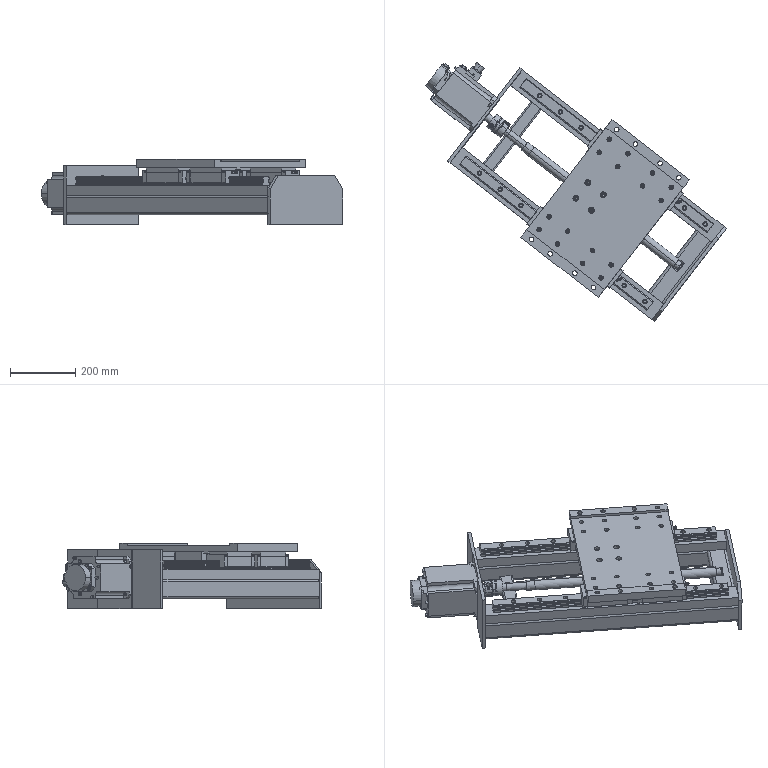Assembly | SolidWorks | mm | 17 component files | 24 solids | 1602 faces | box 920.89 x 791.51 x 200 mm | volume 14788409 mm3 | cylinder 721 | plane 713 | cone 116 | torus 40 | sphere 12 | commonest cylinder face diameters 9 x90 14 x84 0.982 x40 6.8 x40 8.5 x40 5.2 x32 8 x25 5.719 x24
Bill of materials:
0803_Z_Linear_Guide_1 | 2 |  | Long, slender straight bar with a profiled cross-section and a single row of evenly spaced through-holes along its top face; its shape resembles a linear guide rail.
0803_Z_Linear_Guide_2 | 4 |  | Rectangular block with an open channel underneath and a flat top carrying four holes in a rectangular pattern; it has separate end plates and a small nipple-like stud sticking out of one end face. Its shape resembles a linear-guide carriage block.
0803_Z_Servo_Motor_850W_1 | 1 |  | Boxy housing with a square front flange that has chamfered corners and several holes, a raised circular boss with a central bore and a ring of smaller holes, and a rounded rear cap. Small cylindrical protrusions stick out of the side and back. Its overall shape resembles a motor or gearbox housing.
0803_Z_Servo_Motor_850W_2 | 1 |  | Plain solid cylinder with flat ends and no visible features.
0803_205_Plate | 1 |  | Flat rectangular plate with many through-holes of at least two sizes in grouped patterns, raised strips or steps near two edges, and a small step or tab on the underside.
0803_206_Holder | 1 |  | Roughly rectangular block with a large horizontal through-bore and chamfered lower corners. It has four small holes on the top face and four countersunk/conical holes on the opposite face. Its shape resembles a bearing or nut support block.
COLLAR_MISUMI_BSSRK3210-800-F34-P20 | 1 |  | Short thin-walled cylindrical tube (sleeve/ring) with plain ends.
NAT-2_MISUMI_BSSRK3210-800-F34-P20 | 1 |  | Flanged cylindrical body with a central through-bore. The flange is round with two flat sides and has four through-holes plus a small radial hole on its rim. Its shape resembles a flanged nut or bushing.
SHAFT_MISUMI_BSSRK3210-800-F34-P20 | 1 |  | Long, slender stepped round shaft: a main diameter along most of its length, a reduced-diameter section at one end, and a short stepped stub at the other end.
BODY_MISUMI_MCSLC50-24-24_StandardCoupling | 1 |  | Cylindrical body with a central bore that is split by a radial slit at each end, has several partial circumferential slots in the middle, and has radial holes with counterbores. Its shape resembles a slotted, clamp-style flexible shaft coupling.
NEZI-1_MISUMI_MCSLC50-24-24_StandardCoupling | 2 |  | Cap-head screw-like part with a cylindrical head, a hexagonal socket recess, a slightly chamfered head edge, and a plain cylindrical shank.
MotorMountingPlate | 1 |  | Open rectangular frame made of two long parallel side rails joined by end blocks and a cross-bar. One end block has a single round through-hole, and the other end block has chamfered top edges.
Mates:
1. coincident | 0803_102_Servo_Motor_850W-1/0803_Z_Servo_Motor_850W_1-1 face at (-178.235, 965.284, 341.411) dir (0.7899, -0.6132, 0) | MotorMountingPlate-1 face at (-126.114, 1032.428, 241.411) dir (-0.7899, 0.6132, 0)
2. concentric | 0803_102_Servo_Motor_850W-1/0803_Z_Servo_Motor_850W_1-1 face at (-215.723, 912.098, 276.411) dir (-0.7899, 0.6132, 0) r 55 | MotorMountingPlate-1 face at (412.274, 424.608, 276.411) dir (-0.7899, 0.6132, 0) r 55.01
3. parallel | 0803_102_Servo_Motor_850W-1/0803_Z_Servo_Motor_850W_1-1 face at (-178.235, 965.284, 341.411) dir (0.6132, 0.7899, 0) | MotorMountingPlate-1 face at (-176.702, 967.258, 361.411) dir (-0.6132, -0.7899, 0)
4. width | 0803_101_Linear_Guide-1/0803_Z_Linear_Guide_1-1 face at (-88.832, 1025.008, 302.911) dir (0.6132, 0.7899, 0) | 0803_101_Linear_Guide-1/0803_Z_Linear_Guide_1-1 face at (-109.68, 998.15, 302.911) dir (-0.6132, -0.7899, 0) | MotorMountingPlate-1 face at (-101.398, 1051.22, 219.411) dir (0.6132, 0.7899, 0) | MotorMountingPlate-1 face at (-138.19, 1003.824, 263.411) dir (-0.6132, -0.7899, 0)
5. coincident | 0803_101_Linear_Guide-2/0803_Z_Linear_Guide_1-1 face at (-289.04, 767.095, 301.411) dir (0, 0, -1) | MotorMountingPlate-1 face at (472.655, 567.626, 301.411) dir (0, 0, 1)
6. distance | 0803_101_Linear_Guide-1/0803_Z_Linear_Guide_1-1 face at (483.178, 581.183, 327.47) dir (0.7899, -0.6132, 0) | MotorMountingPlate-1 face at (496.353, 549.231, 241.411) dir (-0.7899, 0.6132, 0)
7. concentric | 0803_101_Linear_Guide-1/0803_Z_Linear_Guide_2-1 face at (220.635, 794.908, 356.411) dir (0, 0, 1) r 3.4 | 0803_205_Plate-1 face at (220.635, 794.908, 373.411) dir (0, 0, 1) r 7
8. concentric | 0803_101_Linear_Guide-1/0803_Z_Linear_Guide_2-2 face at (296.469, 736.041, 356.411) dir (0, 0, 1) r 3.4 | 0803_205_Plate-1 face at (296.469, 736.041, 373.411) dir (0, 0, 1) r 7
9. coincident | 0803_205_Plate-1 face at (409.235, 714.967, 356.411) dir (0, 0, -1) | 0803_206_Holder-1 face at (40.67, 647.874, 356.411) dir (0, 0, 1)
10. concentric | 0803_205_Plate-1 face at (109.149, 621.934, 373.411) dir (0, 0, 1) r 9 | 0803_206_Holder-1 face at (109.149, 621.934, 356.411) dir (0, 0, 1) r 4.25
11. concentric | 0803_205_Plate-1 face at (98.545, 706.122, 373.411) dir (0, 0, 1) r 9 | 0803_206_Holder-1 face at (98.545, 706.122, 356.411) dir (0, 0, 1) r 4.25
12. coincident | 0803_101_Linear_Guide-1/0803_Z_Linear_Guide_1-1 face at (-88.733, 1025.136, 327.47) dir (-0.7899, 0.6132, 0) | 0803_101_Linear_Guide-2/0803_Z_Linear_Guide_1-1 face at (-272.691, 788.156, 327.47) dir (-0.7899, 0.6132, 0)
13. width | MotorMountingPlate-1 face at (-285.357, 814.241, 219.411) dir (0.6132, 0.7899, 0) | MotorMountingPlate-1 face at (-322.148, 766.845, 263.411) dir (-0.6132, -0.7899, 0) | 0803_101_Linear_Guide-2/0803_Z_Linear_Guide_1-1 face at (-293.639, 761.171, 302.911) dir (-0.6132, -0.7899, 0) | 0803_101_Linear_Guide-2/0803_Z_Linear_Guide_1-1 face at (-272.79, 788.028, 302.911) dir (0.6132, 0.7899, 0)
14. concentric | 0803_101_Linear_Guide-2/0803_Z_Linear_Guide_2-1 face at (-20.198, 602.078, 338.161) dir (0, 0, -1) r 1029.744 | 0803_205_Plate-1 face at (-20.198, 602.078, 373.411) dir (0, 0, 1) r 4.5
15. concentric | 0803_101_Linear_Guide-2/0803_Z_Linear_Guide_2-1 face at (-50.858, 562.582, 356.411) dir (0, 0, 1) r 3.4 | 0803_205_Plate-1 face at (-50.858, 562.582, 373.411) dir (0, 0, 1) r 7
16. coincident | 0803_101_Linear_Guide-1/0803_Z_Linear_Guide_1-1 face at (-90.656, 1022.658, 327.411) dir (0, 0, 1) | 0803_101_Linear_Guide-2/0803_Z_Linear_Guide_1-1 face at (-274.615, 785.678, 327.411) dir (0, 0, 1)
17. concentric | 0803_101_Linear_Guide-2/0803_Z_Linear_Guide_2-2 face at (169.386, 454.912, 356.411) dir (0, 0, 1) r 3.4 | 0803_205_Plate-1 face at (169.386, 454.912, 373.411) dir (0, 0, 1) r 7
18. coincident | 0803_101_Linear_Guide-2/0803_Z_Linear_Guide_2-2 face at (44.122, 476.193, 356.411) dir (0, 0, 1) | 0803_205_Plate-1 face at (199.216, 444.415, 356.411) dir (0, 0, -1)
19. concentric | 0803_102_Servo_Motor_850W-1/0803_Z_Servo_Motor_850W_2-1 face at (-231.001, 923.958, 276.411) dir (-0.7899, 0.6132, 0) r 12 | MISUMI_BSSRK3210-800-F34-P20-1/SHAFT_MISUMI_BSSRK3210-800-F34-P20-1 face at (382.255, 447.91, 276.411) dir (0.7899, -0.6132, 0) r 16
20. concentric | 0803_206_Holder-1 face at (135.445, 639.5, 276.411) dir (-0.7899, 0.6132, 0) r 33.5 | MISUMI_BSSRK3210-800-F34-P20-1/NAT-2_MISUMI_BSSRK3210-800-F34-P20-1 face at (133.075, 641.34, 276.411) dir (0.7899, -0.6132, 0) r 33.5
21. coincident | 0803_206_Holder-1 face at (40.67, 647.874, 233.911) dir (-0.7899, 0.6132, 0) | MISUMI_BSSRK3210-800-F34-P20-1/NAT-2_MISUMI_BSSRK3210-800-F34-P20-1 face at (40.67, 647.874, 276.411) dir (0.7899, -0.6132, 0)
22. concentric | 0803_206_Holder-1 face at (49.681, 659.481, 255.161) dir (-0.7899, 0.6132, 0) r 3.4 | MISUMI_BSSRK3210-800-F34-P20-1/NAT-2_MISUMI_BSSRK3210-800-F34-P20-1 face at (37.832, 668.679, 255.161) dir (0.7899, -0.6132, 0) r 4.5
23. distance | MISUMI_BSSRK3210-800-F34-P20-1/SHAFT_MISUMI_BSSRK3210-800-F34-P20-1 face at (-170.697, 877.146, 276.411) dir (-0.7899, 0.6132, 0) | 0803_102_Servo_Motor_850W-1/0803_Z_Servo_Motor_850W_2-1 face at (-174.647, 880.212, 276.411) dir (0.7899, -0.6132, 0)
24. coincident | 0803_102_Servo_Motor_850W-1/0803_Z_Servo_Motor_850W_1-1 face at (-178.235, 965.284, 341.411) dir (0.7899, -0.6132, 0) | MotorMountingPlate-1 face at (-126.114, 1032.428, 241.411) dir (-0.7899, 0.6132, 0)
25. concentric | MISUMI_BSSRK3210-800-F34-P20-1/SHAFT_MISUMI_BSSRK3210-800-F34-P20-1 face at (382.255, 447.91, 276.411) dir (0.7899, -0.6132, 0) r 12.5 | MISUMI_MCSLC50-24-24_StandardCoupling-1/BODY_MISUMI_MCSLC50-24-24_StandardCoupling-1 face at (-181.835, 885.792, 276.411) dir (-0.7899, 0.6132, 0) r 12
26. distance | MISUMI_MCSLC50-24-24_StandardCoupling-1/BODY_MISUMI_MCSLC50-24-24_StandardCoupling-1 face at (-196.054, 896.83, 276.411) dir (-0.7899, 0.6132, 0) | 0803_102_Servo_Motor_850W-1/0803_Z_Servo_Motor_850W_1-1 face at (-215.802, 912.16, 276.411) dir (0.7899, -0.6132, 0)
27. coincident | 0803_Z_Linear_Guide_1-1 face at (14.024, 724, 0) dir (0, 0, 1) | 0803_Z_Linear_Guide_2-1 face at (-14.024, 729.245, 0) dir (0, 0, -1)
28. width | 0803_Z_Linear_Guide_2-1 face at (34.5, 729.245, -17) dir (1, 0, 0) | 0803_Z_Linear_Guide_2-1 face at (-34.5, 729.245, -17) dir (-1, 0, 0) | 0803_Z_Linear_Guide_1-1 face at (-17, 724, -24.5) dir (-1, 0, 0) | 0803_Z_Linear_Guide_1-1 face at (17, 724, -24.5) dir (1, 0, 0)
29. coincident | 0803_Z_Linear_Guide_2-1 face at (34.5, 729.245, -17) dir (1, 0, 0) | 0803_Z_Linear_Guide_2-2 face at (34.5, 423.994, -17) dir (1, 0, 0)
30. coincident | 0803_Z_Linear_Guide_2-1 face at (-35, 729.245, 29) dir (0, 0, 1) | 0803_Z_Linear_Guide_2-2 face at (-35, 423.994, 29) dir (0, 0, 1)
31. concentric | 0803_Z_Servo_Motor_850W_1-1 face at (0, 148.5, 0) dir (0, 1, 0) r 12 | 0803_Z_Servo_Motor_850W_2-1 face at (0, 137.159, 0) dir (0, -1, 0) r 12
32. coincident | 0803_Z_Servo_Motor_850W_1-1 face at (0, 148.5, 0) dir (0, 1, 0) | 0803_Z_Servo_Motor_850W_2-1 face at (0, 148.5, 0) dir (0, -1, 0)
33. coincident | SHAFT_MISUMI_BSSRK3210-800-F34-P20-1 face at (579, 12.5, 0) dir (1, 0, 0) | COLLAR_MISUMI_BSSRK3210-800-F34-P20-1 face at (579, 15.5, 0) dir (-1, 0, 0)
34. coincident | ref31-1 plane at (104.5, 0, 0) dir (0, 0, 1) | MISUMI_BSSRK3210-800-F34-P20 plane at (0, 0, 0) dir (0, 0, 1)
35. coincident | COLLAR_MISUMI_BSSRK3210-800-F34-P20-1 plane at (579, 0, 0) dir (0, 0, 1) | MISUMI_BSSRK3210-800-F34-P20 plane at (0, 0, 0) dir (0, 0, 1)
36. coincident | ref31-2 plane at (63.5, 0, 0) dir (0, 0, -1) | MISUMI_BSSRK3210-800-F34-P20 plane at (0, 0, 0) dir (0, 0, 1)
37. coincident | NAT-2_MISUMI_BSSRK3210-800-F34-P20-1 plane at (392.446, 0, 0) dir (0, 0, 1) | MISUMI_BSSRK3210-800-F34-P20 plane at (0, 0, 0) dir (0, 0, 1)
38. coincident | NAT-2_MISUMI_BSSRK3210-800-F34-P20-2 plane at (69, 0, 0) dir (0, 0, -1) | MISUMI_BSSRK3210-800-F34-P20 plane at (0, 0, 0) dir (0, 0, 1)
39. coincident | ref32-1 plane at (128, 0, 0) dir (0, 0, 1) | MISUMI_BSSRK3210-800-F34-P20 plane at (0, 0, 0) dir (0, 0, 1)
40. coincident | ref32-2 plane at (72, 0, 0) dir (0, 0, -1) | MISUMI_BSSRK3210-800-F34-P20 plane at (0, 0, 0) dir (0, 0, 1)
41. coincident | SHAFT_MISUMI_BSSRK3210-800-F34-P20-1 face at (700, 0, 0) dir (1, 0, 0) | COLLAR_MISUMI_BSSRK3210-800-F34-P20-2 face at (800, 15.5, 0) dir (-1, 0, 0)
42. concentric | SHAFT_MISUMI_BSSRK3210-800-F34-P20-1 face at (0, 0, 0) dir (-1, 0, 0) r 16 | ref31-1 face at (51.5, 0, 0) dir (-1, 0, 0) r 14
43. concentric | SHAFT_MISUMI_BSSRK3210-800-F34-P20-1 face at (0, 0, 0) dir (-1, 0, 0) r 12.5 | COLLAR_MISUMI_BSSRK3210-800-F34-P20-1 face at (579, 0, 0) dir (-1, 0, 0) r 12.5
44. concentric | SHAFT_MISUMI_BSSRK3210-800-F34-P20-1 face at (0, 0, 0) dir (-1, 0, 0) r 16 | ref31-2 face at (116.5, 0, 0) dir (1, 0, 0) r 14
45. concentric | SHAFT_MISUMI_BSSRK3210-800-F34-P20-1 face at (0, 0, 0) dir (-1, 0, 0) r 16 | NAT-2_MISUMI_BSSRK3210-800-F34-P20-1 face at (315.446, 0, 0) dir (-1, 0, 0) r 16
46. concentric | NAT-2_MISUMI_BSSRK3210-800-F34-P20-2 face at (146, 0, 0) dir (1, 0, 0) r 16 | SHAFT_MISUMI_BSSRK3210-800-F34-P20-1 face at (0, 0, 0) dir (-1, 0, 0) r 16
47. concentric | SHAFT_MISUMI_BSSRK3210-800-F34-P20-1 face at (0, 0, 0) dir (-1, 0, 0) r 16 | ref32-1 face at (57, 0, 0) dir (-1, 0, 0) r 16
48. concentric | SHAFT_MISUMI_BSSRK3210-800-F34-P20-1 face at (0, 0, 0) dir (-1, 0, 0) r 16 | ref32-2 face at (143, 0, 0) dir (1, 0, 0) r 16
49. concentric | SHAFT_MISUMI_BSSRK3210-800-F34-P20-1 face at (0, 0, 0) dir (-1, 0, 0) r 16 | COLLAR_MISUMI_BSSRK3210-800-F34-P20-2 face at (800, 0, 0) dir (-1, 0, 0) r 12.5
50. coincident | BODY_MISUMI_MCSLC50-24-24_StandardCoupling-1 face at (12.3, -17.247, 5.518) dir (0, -0.08716, 0.9962) | NEZI-1_MISUMI_MCSLC50-24-24_StandardCoupling-1 face at (9, -14.258, 5.779) dir (0, 0.08716, -0.9962)
51. coincident | BODY_MISUMI_MCSLC50-24-24_StandardCoupling-1 face at (47.3, 17.247, 5.518) dir (0, 0.08716, 0.9962) | NEZI-1_MISUMI_MCSLC50-24-24_StandardCoupling-2 face at (44, 20.235, 5.256) dir (0, -0.08716, -0.9962)
52. concentric | BODY_MISUMI_MCSLC50-24-24_StandardCoupling-1 face at (9, -18.815, 23.449) dir (0, -0.08716, 0.9962) r 3.3 | NEZI-1_MISUMI_MCSLC50-24-24_StandardCoupling-1 face at (9, -17.754, 11.316) dir (0, -0.08716, 0.9962) r 3
53. concentric | BODY_MISUMI_MCSLC50-24-24_StandardCoupling-1 face at (44, 18.815, 23.449) dir (0, 0.08716, 0.9962) r 3.3 | NEZI-1_MISUMI_MCSLC50-24-24_StandardCoupling-2 face at (44, 17.754, 11.316) dir (0, 0.08716, 0.9962) r 3
54. parallel | NEZI-1_MISUMI_MCSLC50-24-24_StandardCoupling-1 plane at (9, -17.247, 5.518) dir (1, 0, 0) | MISUMI_MCSLC50-24-24_StandardCoupling plane at (0, 0, 0) dir (1, 0, 0)
55. parallel | NEZI-1_MISUMI_MCSLC50-24-24_StandardCoupling-2 plane at (44, 17.247, 5.518) dir (1, 0, 0) | MISUMI_MCSLC50-24-24_StandardCoupling plane at (0, 0, 0) dir (1, 0, 0)